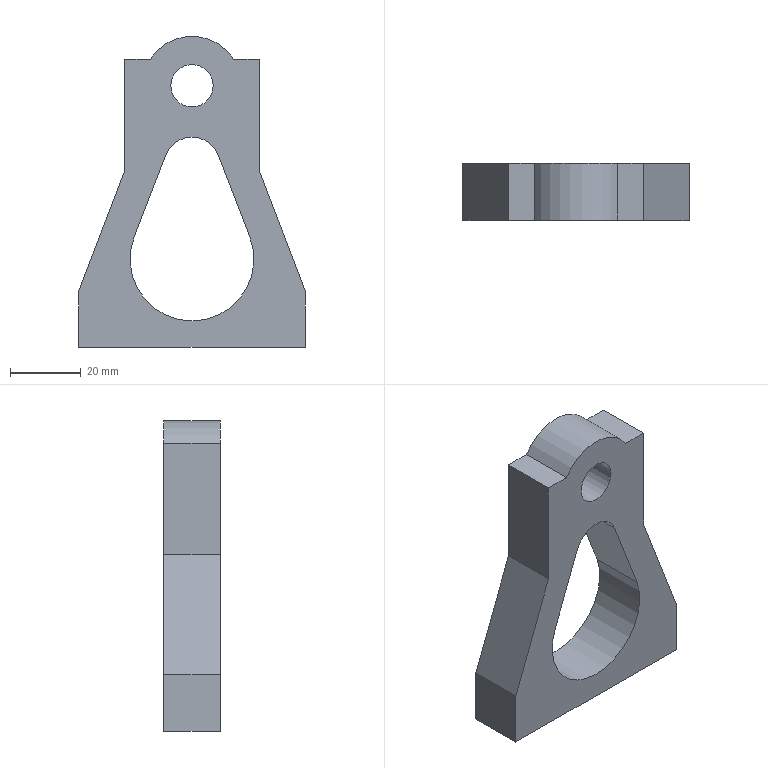Component | NX | BRACKET_3 | 1 solid | 23 faces | volume 41890 mm3 | plane 13 | cylinder 6 | cone 4 | commonest cylinder face diameters 5 x2 35 x1 16 x1 28 x1 12 x1